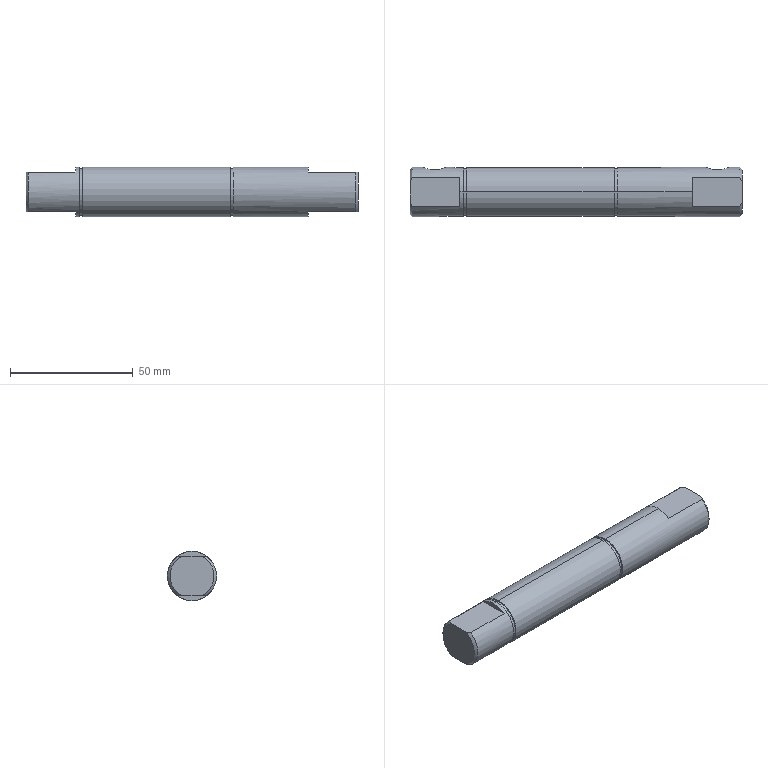Component | SolidWorks | J-TRD899MINI-2213-04PressingWheelAxis-1 | 1 solid | 34 faces | box 135 x 20 x 20 mm | volume 40621 mm3 | plane 16 | cylinder 14 | cone 4 | commonest cylinder face diameters 20 x6 9 x4 19 x4 | material 45
build123d program:
from build123d import *

# Parameters (mm, degrees)
SKETCH1_W               = 135
SKETCH1_H               = 10
CHAMFER1_SIZE           = 1
CUT_EXTRUDE1_DEPTH      = 136.739
CUT_EXTRUDE1_DEPTH_BACK = 136.739
SKETCH2_W               = 2
SKETCH2_H               = 20.2
SKETCH4_R               = 4.5
CUT_EXTRUDE2_DEPTH      = 3
SKETCH5_W               = 1.35
SKETCH5_H               = 0.5


with BuildPart() as part:
    # Sketch1 → Revolve1 (revolve)
    with BuildSketch(Plane(origin=(0, 0, 0), x_dir=(0, 0, -1), z_dir=(1, 0, 0)), mode=Mode.PRIVATE) as revolve1_sk:
        with Locations((67.5, 5)):
            Rectangle(SKETCH1_W, SKETCH1_H)
    revolve(revolve1_sk.sketch.rotate(Axis((0, 0, 0), (0, 0, -1)), 90), axis=Axis((0, 0, 0), (0, 0, -1)))

    # Chamfer1
    chamfer1_edges = [part.edges().sort_by_distance(p)[0] for p in [
        (-10, 0, -135),
        (-10, 0, 0),
    ]]
    chamfer(chamfer1_edges, length=CHAMFER1_SIZE)

    # Sketch2 → Cut-Extrude1 (cut, two sides: drawn at the far end of the back side and taken through both)
    with BuildSketch(Plane(origin=(0, 0, 0), x_dir=(1, 0, 0), z_dir=(0, 1, 0)).offset(-CUT_EXTRUDE1_DEPTH_BACK)):
        with Locations((-9, 124.9)):
            Rectangle(SKETCH2_W, SKETCH2_H)
        with Locations((9, 124.9)):
            Rectangle(SKETCH2_W, SKETCH2_H)
        with Locations((9, 10.1)):
            Rectangle(SKETCH2_W, SKETCH2_H)
        with Locations((-9, 10.1)):
            Rectangle(SKETCH2_W, SKETCH2_H)
    extrude(amount=CUT_EXTRUDE1_DEPTH + CUT_EXTRUDE1_DEPTH_BACK, mode=Mode.SUBTRACT)

    # Sketch4 → Cut-Extrude2 (cut)
    with BuildSketch(Plane(origin=(0, 10, 0), x_dir=(1, 0, 0), z_dir=(0, 1, 0))):
        with Locations(Location((0, 125, 0), (0, 0, 270))):
            Circle(SKETCH4_R)
        with Locations(Location((0, 10, 0), (0, 0, 270))):
            Circle(SKETCH4_R)
    extrude(amount=-CUT_EXTRUDE2_DEPTH, mode=Mode.SUBTRACT)

    # Sketch5 → Cut-Revolve1 (revolve, cut)
    with BuildSketch(Plane(origin=(0, 0, 0), x_dir=(0, 0, -1), z_dir=(1, 0, 0)), mode=Mode.PRIVATE) as cut_revolve1_sk:
        with Locations((112.675, 9.75)):
            Rectangle(SKETCH5_W, SKETCH5_H)
        with Locations((51.325, 9.75)):
            Rectangle(SKETCH5_W, SKETCH5_H)
    revolve(cut_revolve1_sk.sketch.rotate(Axis((0, 0, 0), (0, 0, -1)), 90), axis=Axis((0, 0, 0), (0, 0, -1)), mode=Mode.SUBTRACT)


solid = part.part

# Placed as in the assembly
solid = solid.moved(Location((3.337, 20.996, 191.6), (0, 90, 0)))